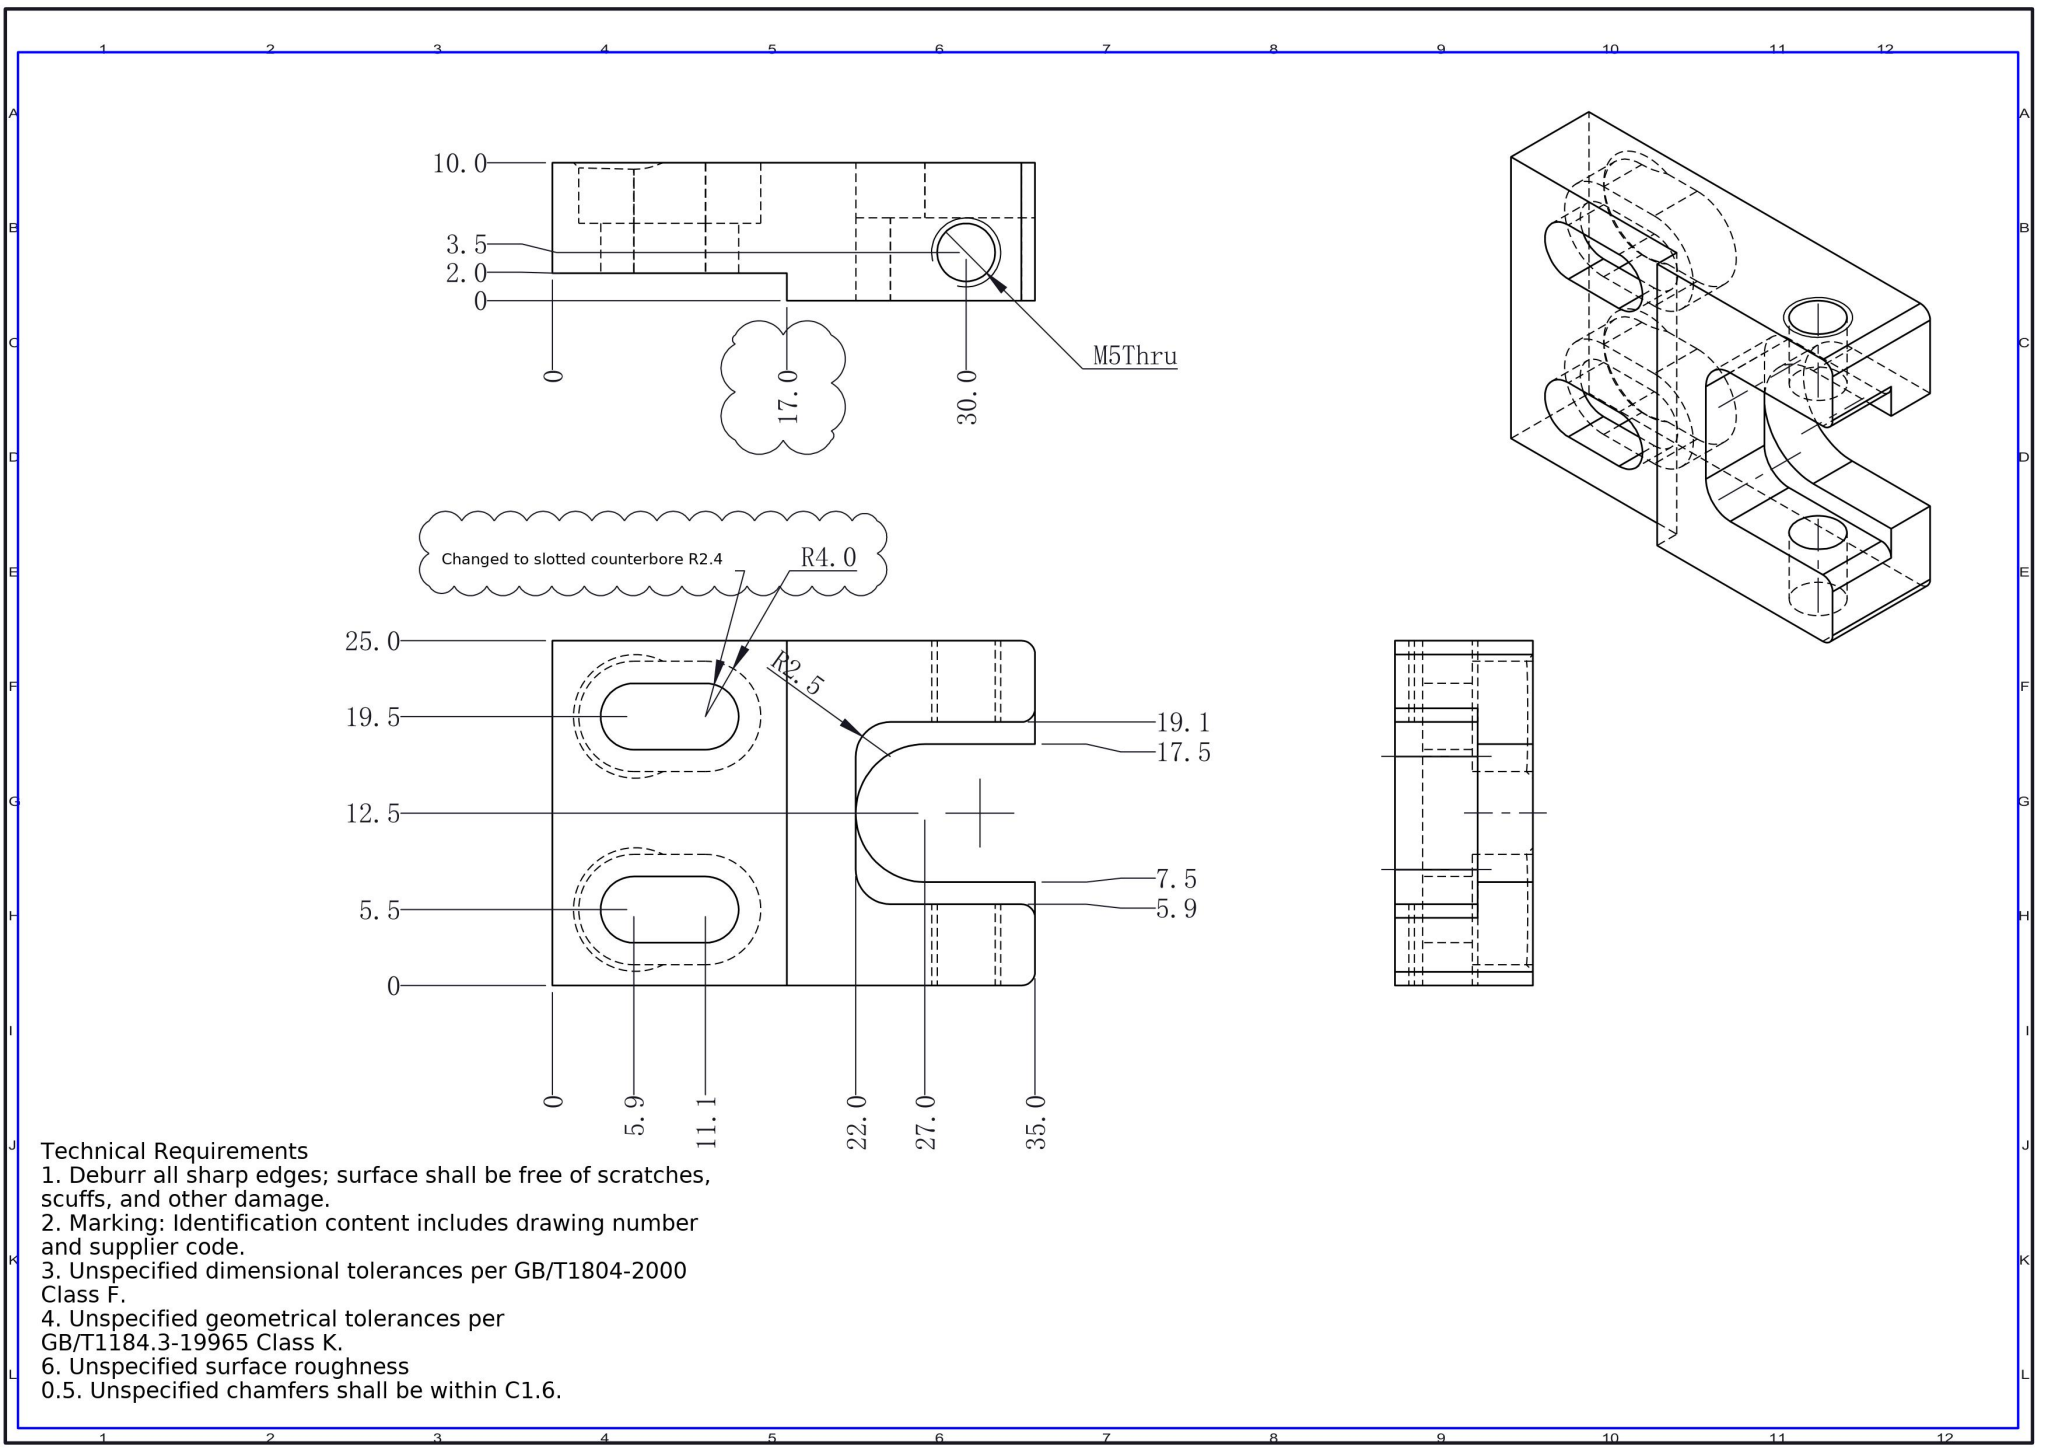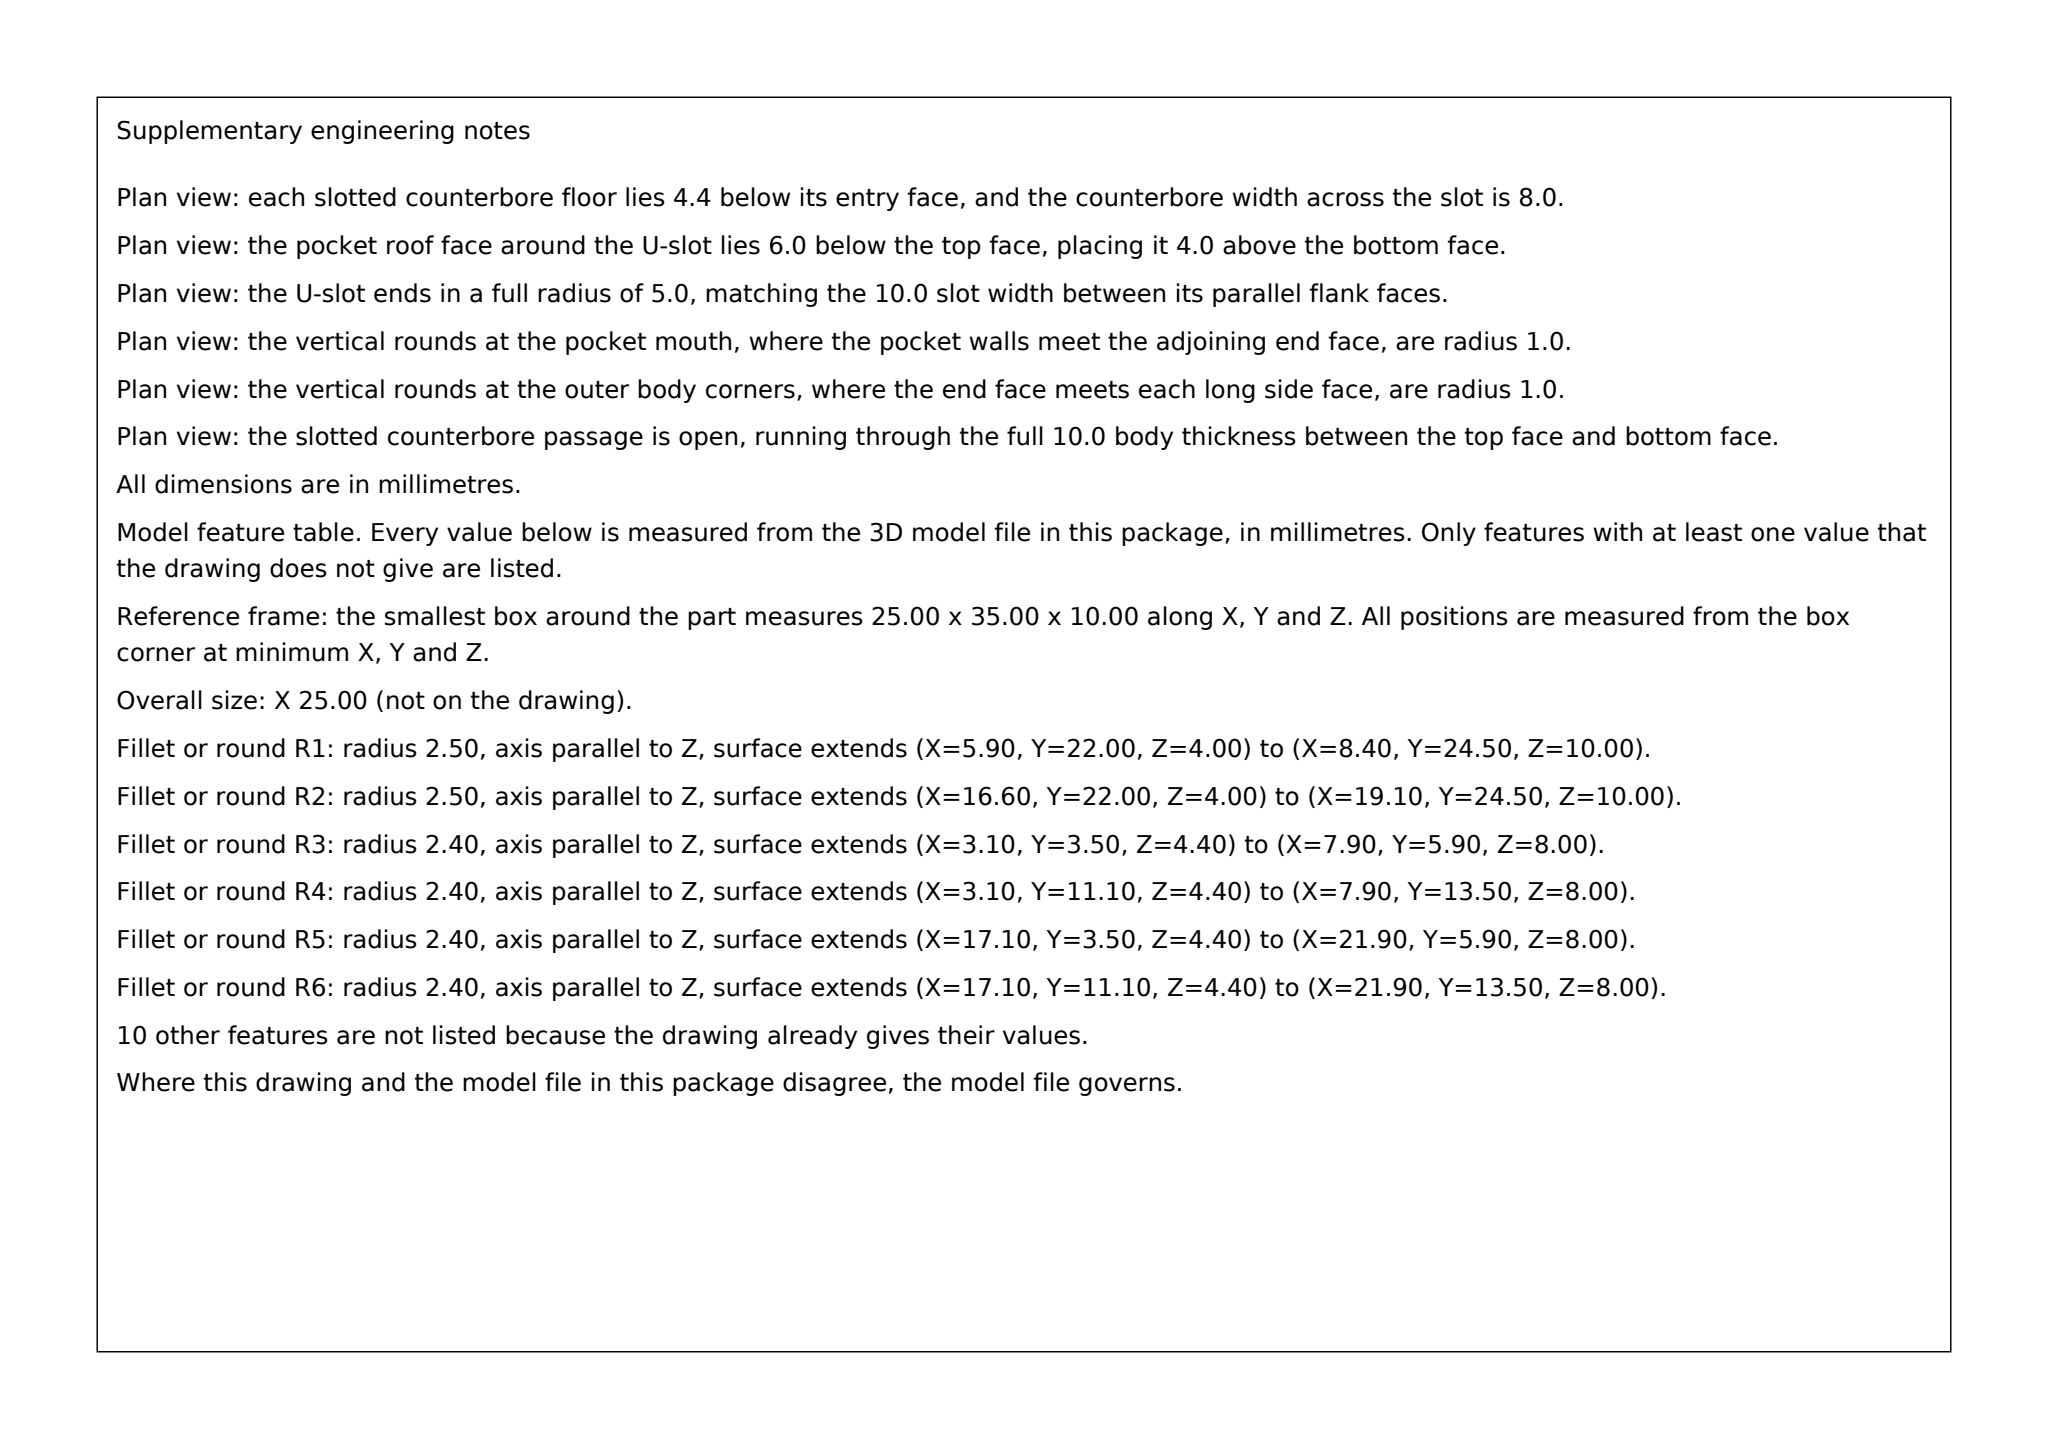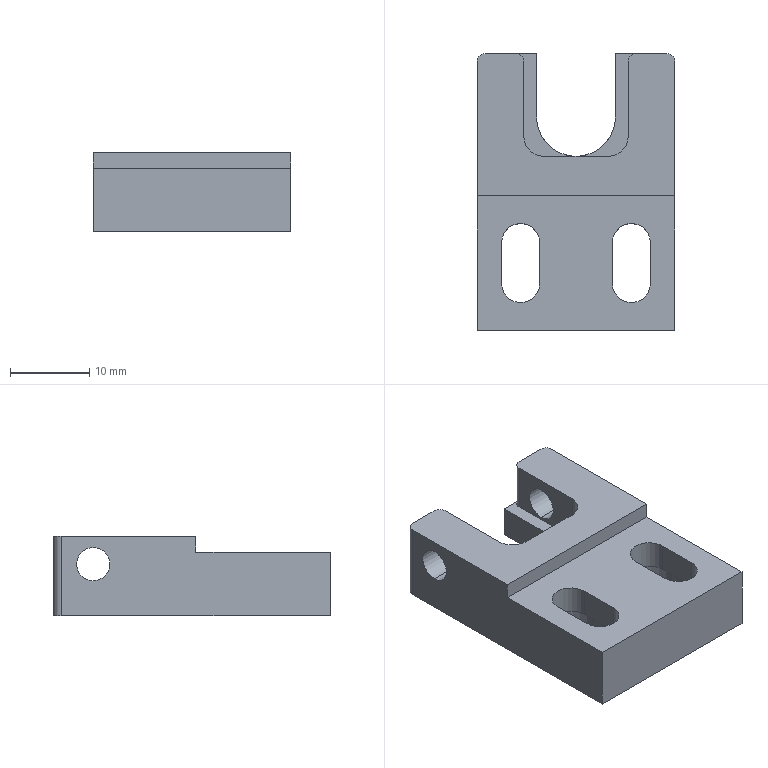Part | SolidWorks | mm | 1 solid | 51 faces | box 25 x 35 x 10 mm | volume 5118 mm3 | plane 26 | cylinder 19 | cone 6 | commonest cylinder face diameters 4.2 x4 2 x4 8 x4 4.8 x4 5 x2 10 x1